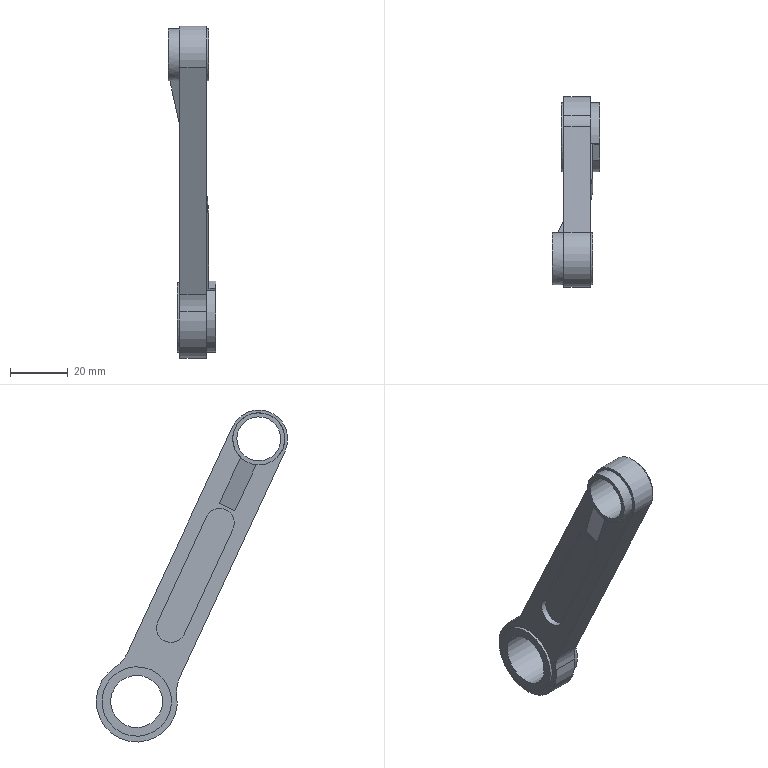Component | NX | LINK_ROD | 1 solid | 31 faces | volume 19399 mm3 | plane 19 | cylinder 12 | commonest cylinder face diameters 18 x3 20 x3 24 x2 10 x2 15.2 x1 28 x1